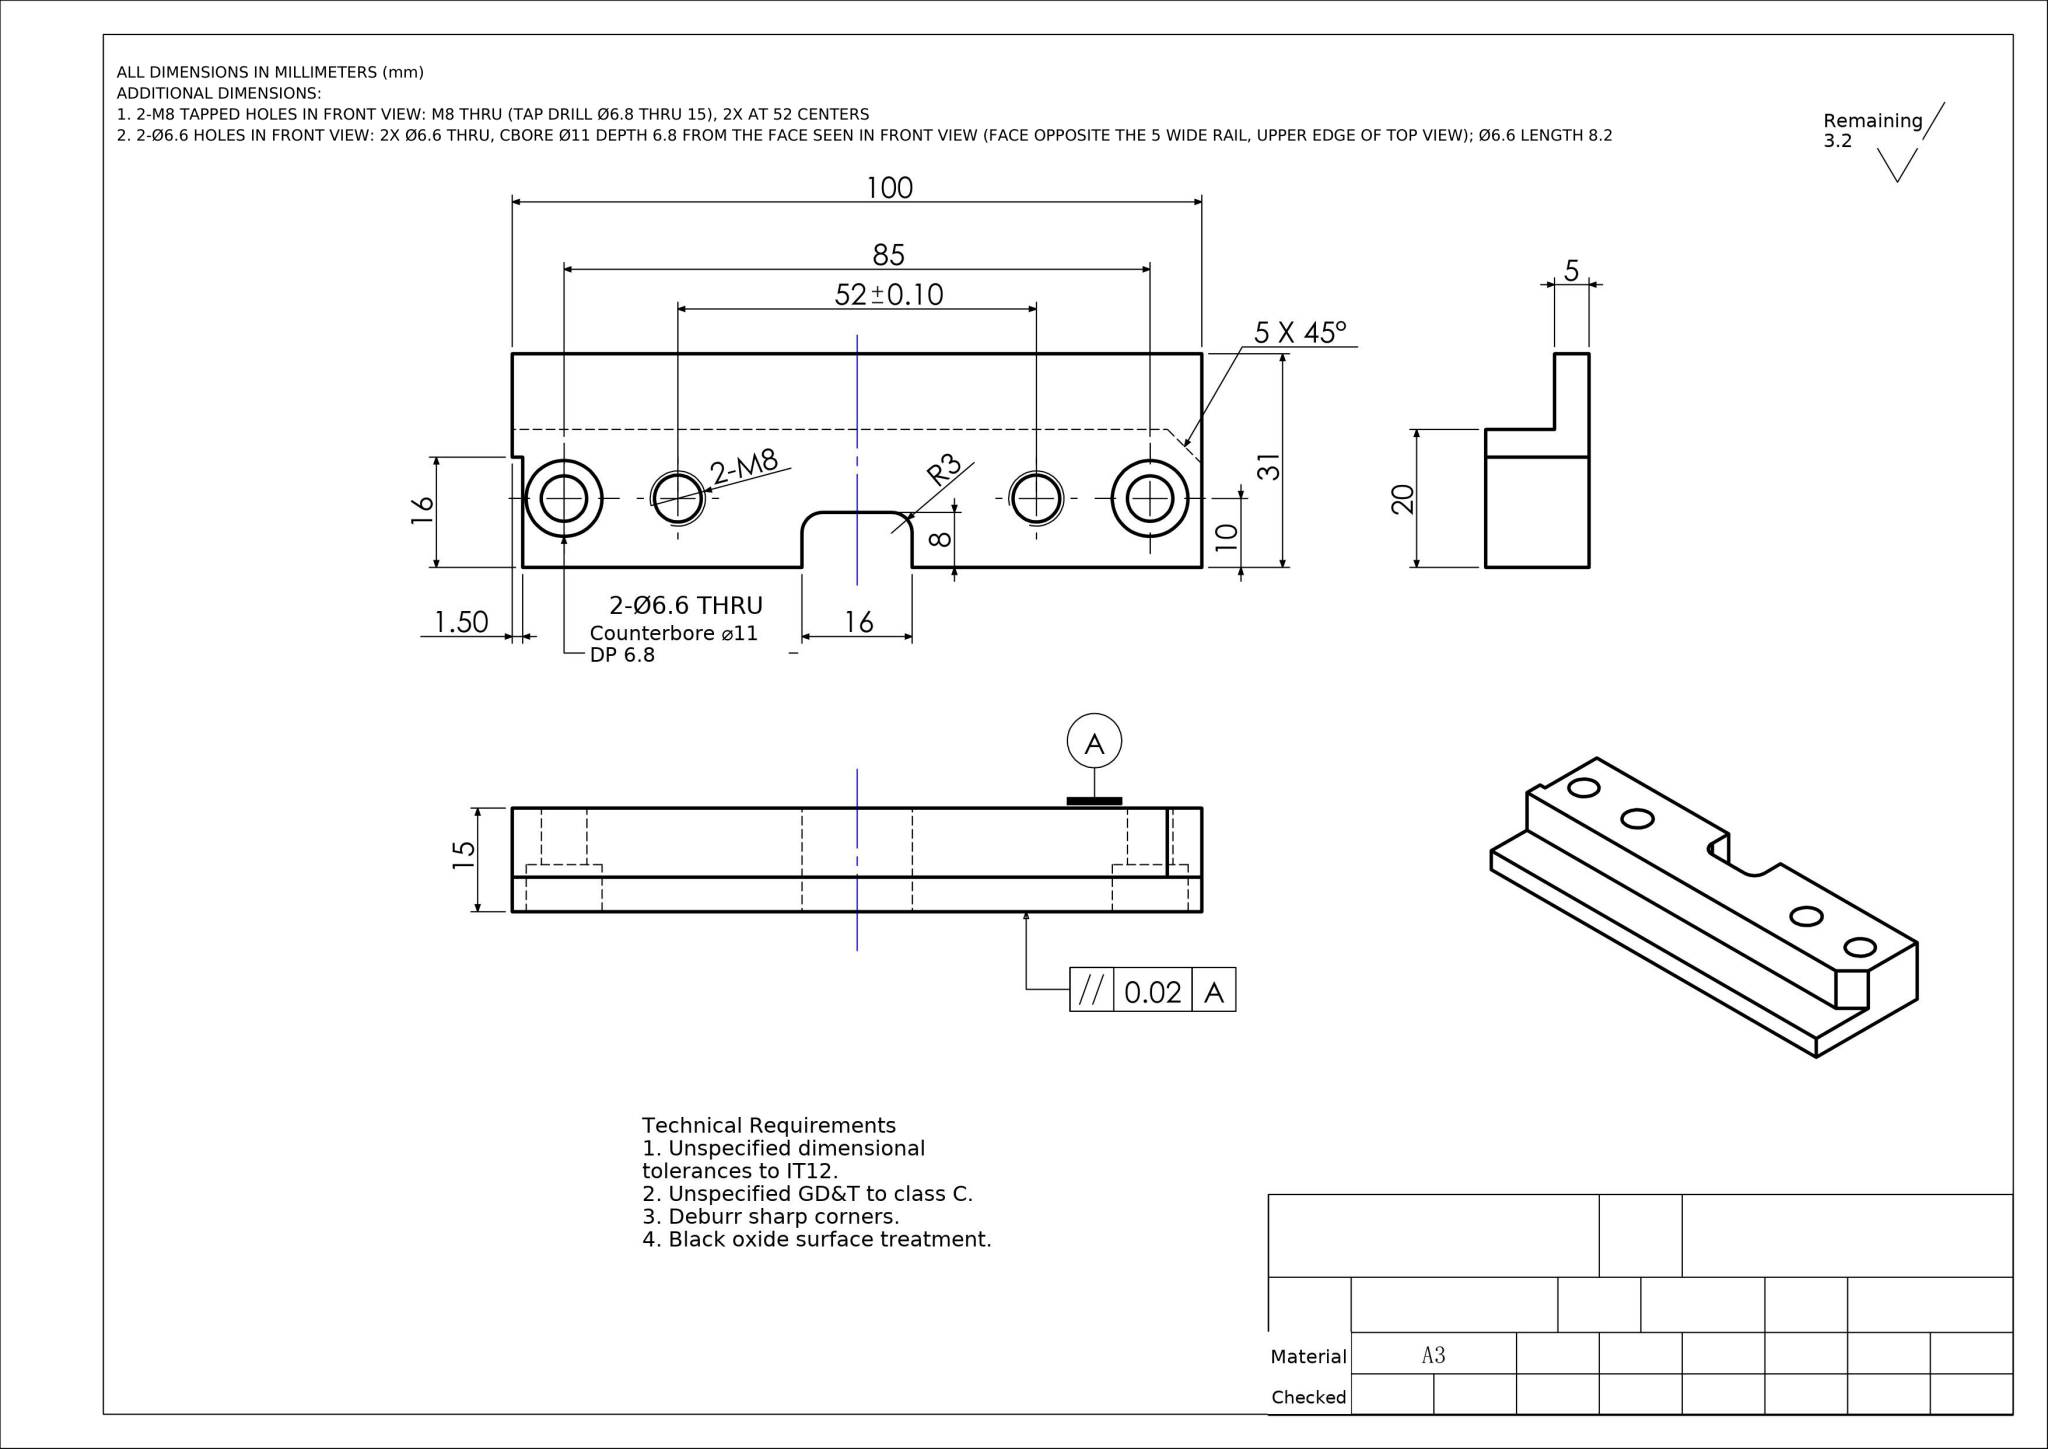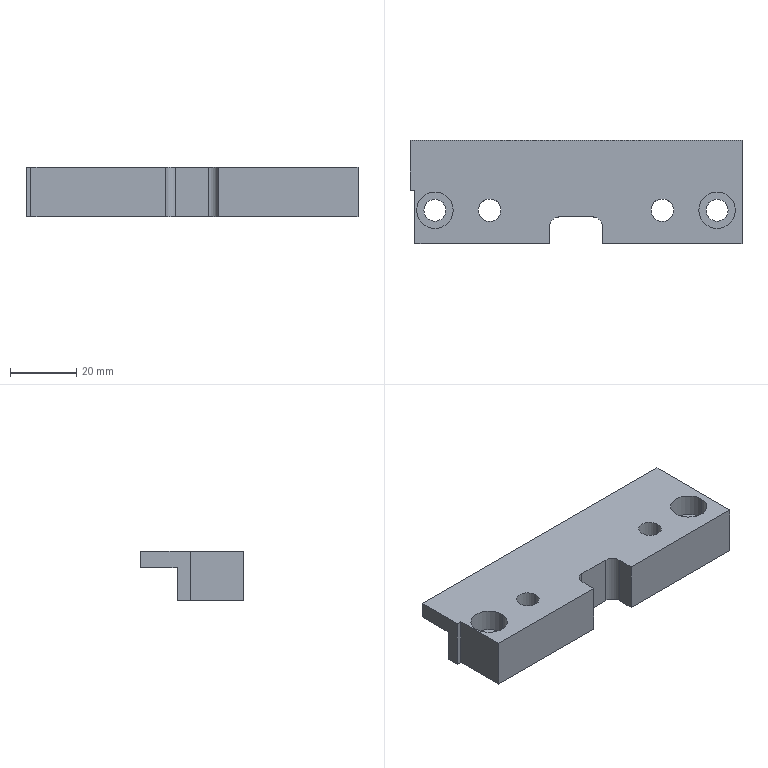Part | NX | mm | 1 solid | 31 faces | box 100 x 31 x 15 mm | volume 30210 mm3 | plane 17 | cylinder 14 | commonest cylinder face diameters 6.8 x4 11 x4 6.6 x4 6 x2